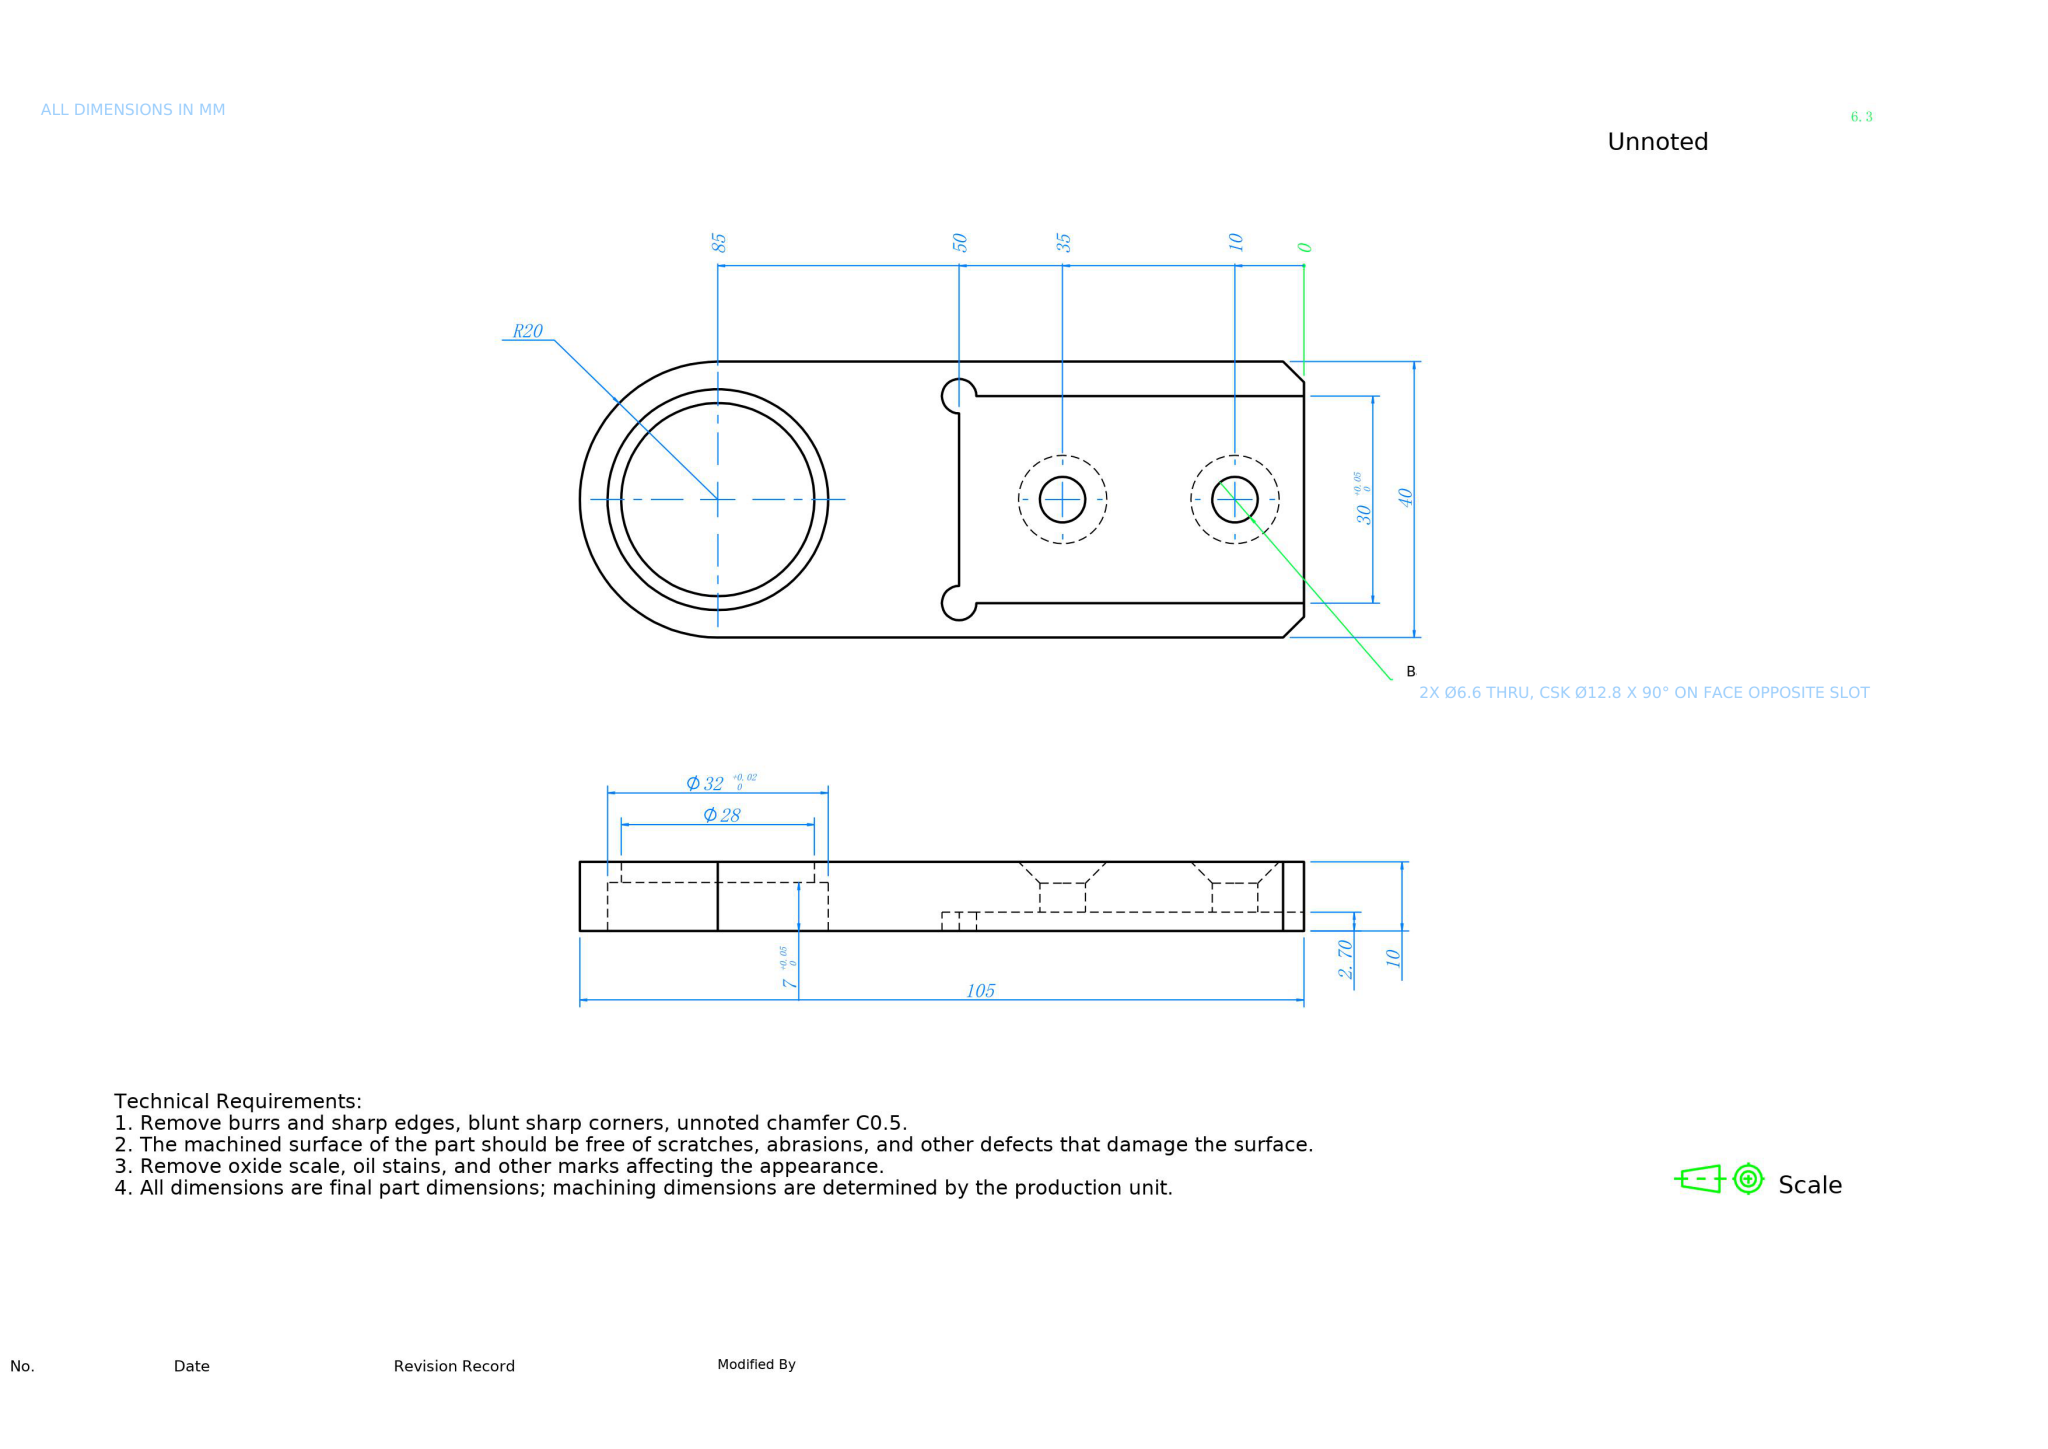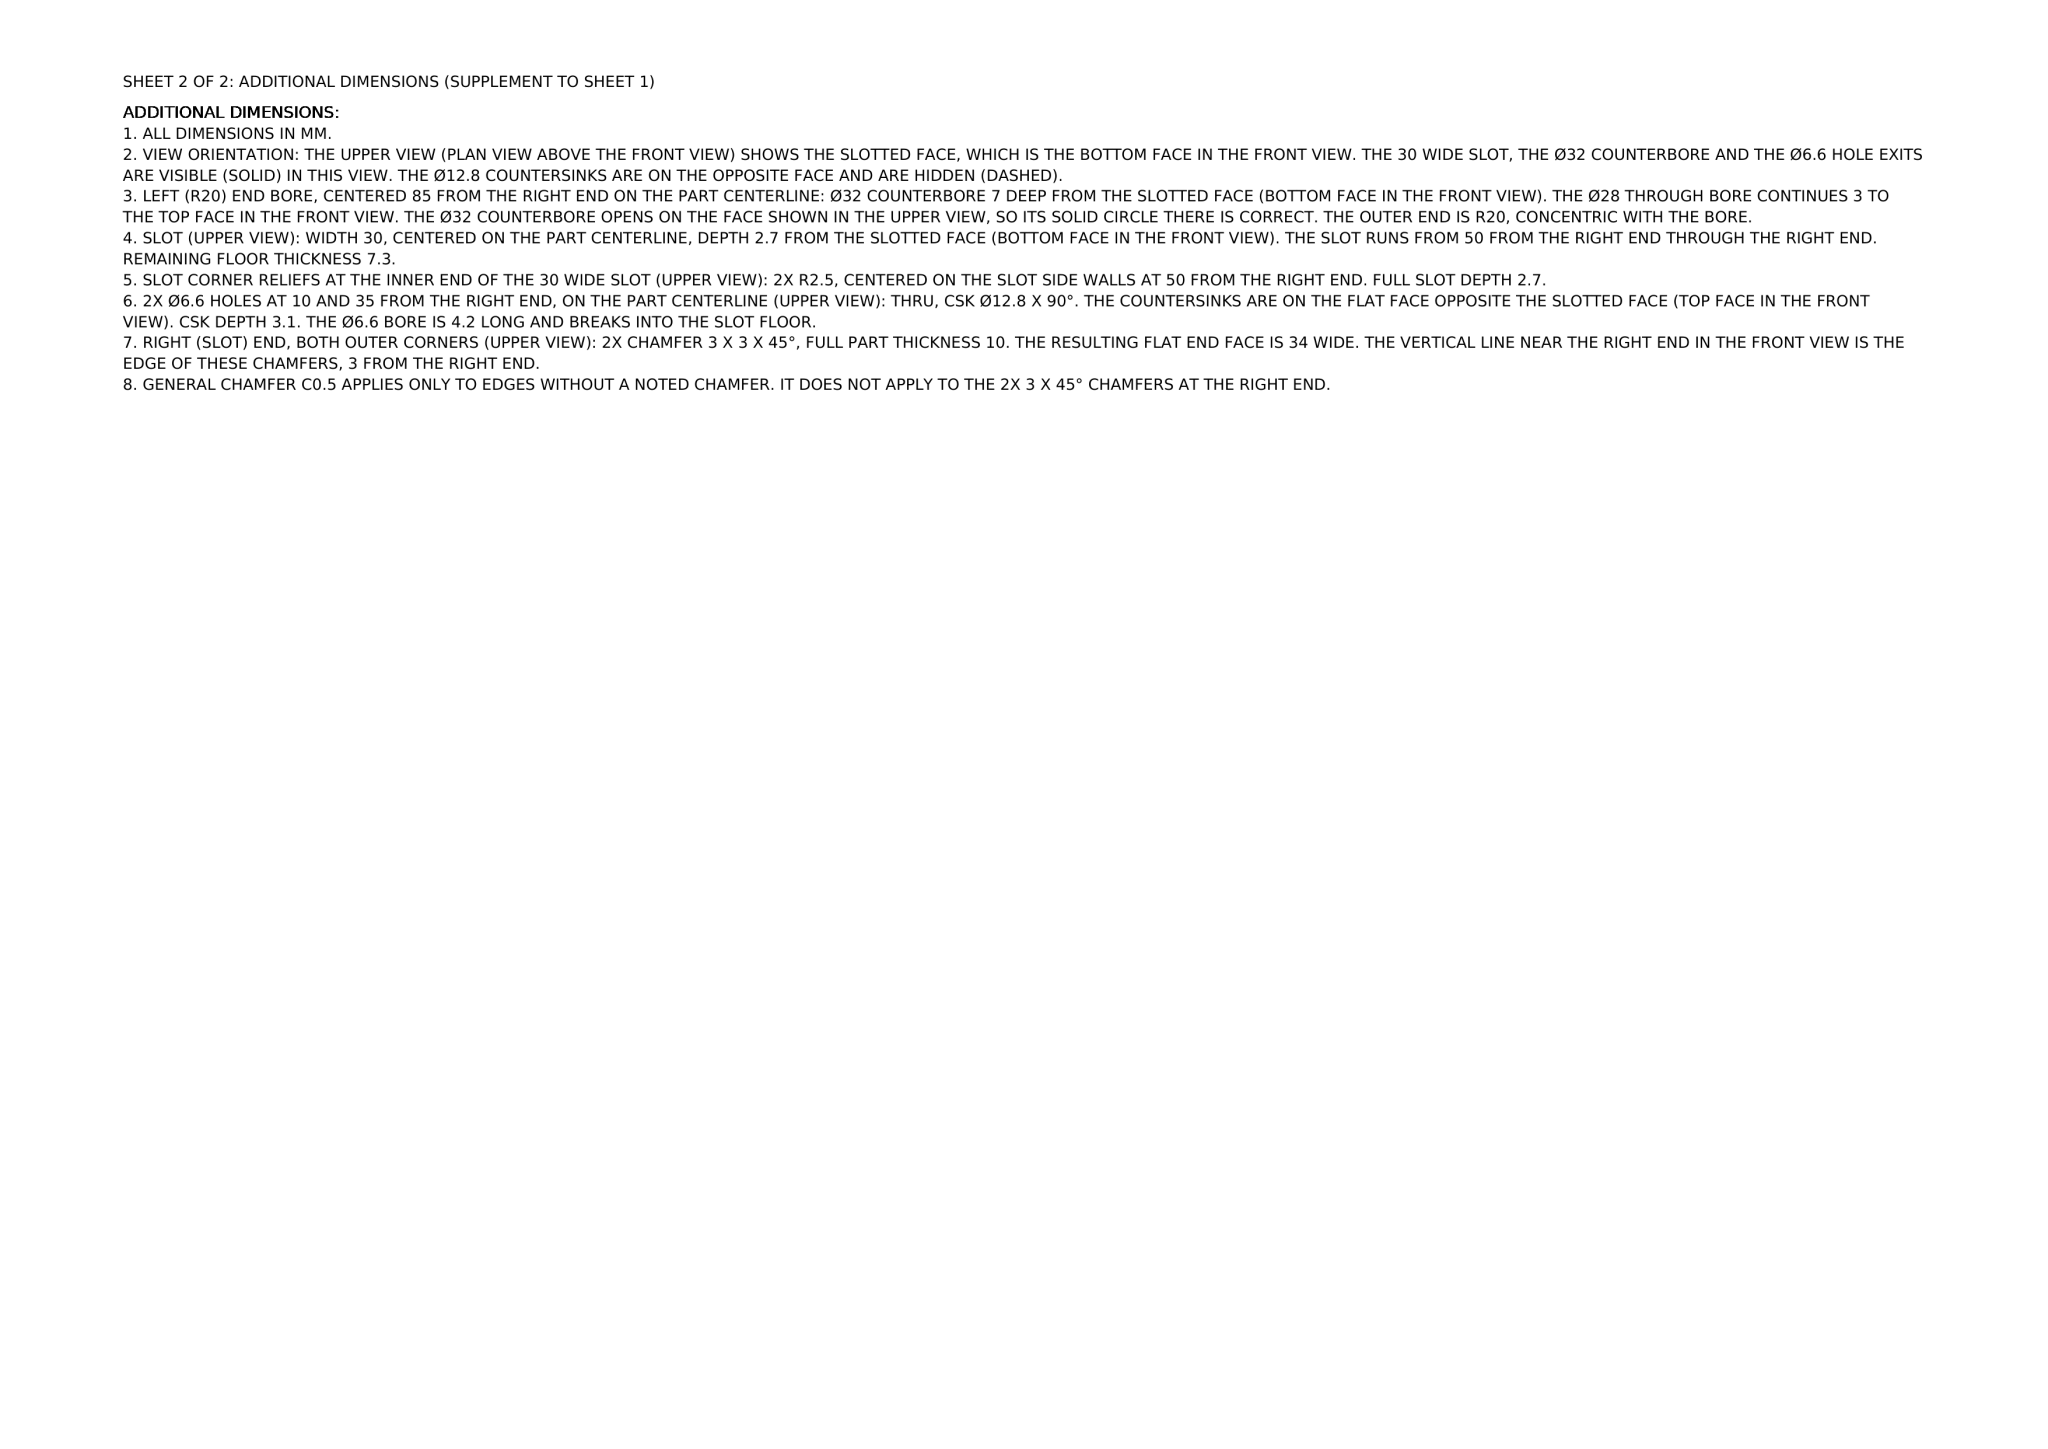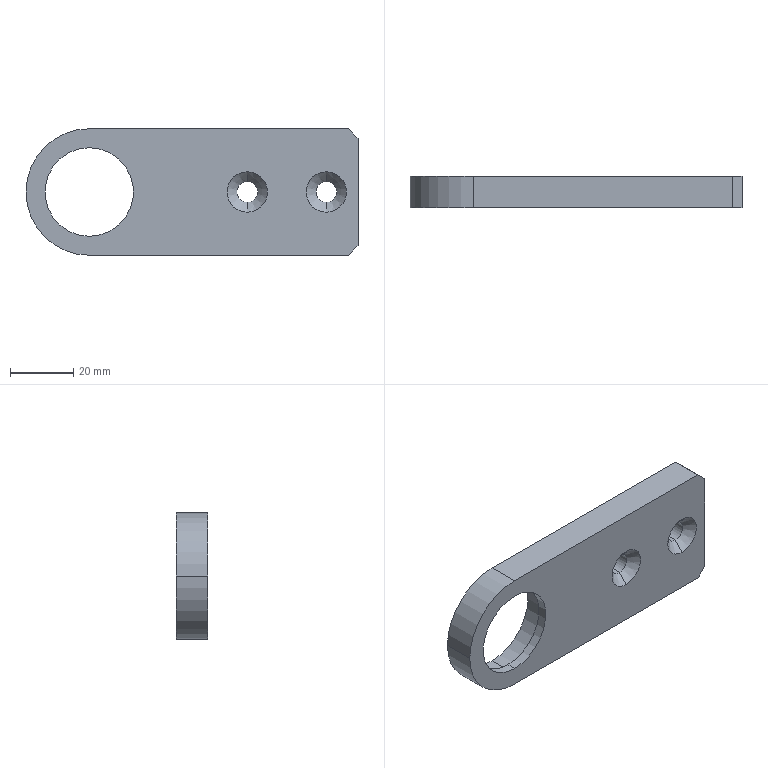Part | NX | mm | 1 solid | 29 faces | box 105 x 10 x 40 mm | volume 27826 mm3 | cylinder 13 | plane 12 | cone 4 | commonest cylinder face diameters 6.6 x4 5 x3 28 x2 32 x2 40 x2